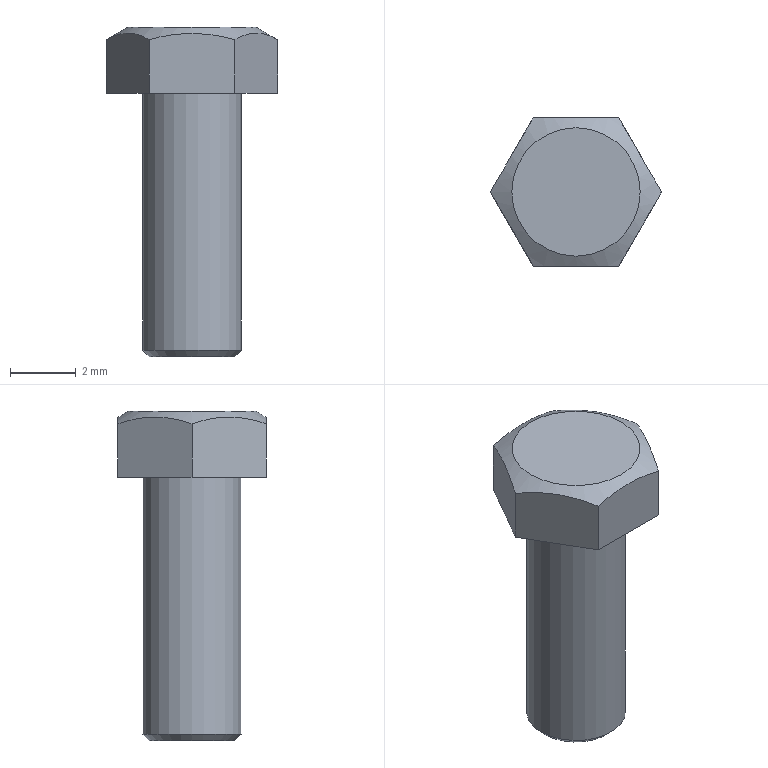Component | NX | SCREW_M3X8 | 1 solid | 12 faces | box 5.2 x 4.5 x 10 mm | volume 91 mm3 | plane 9 | cone 2 | cylinder 1 | commonest cylinder face diameters 3 x1
STEP:
#1=CARTESIAN_POINT('',(0.,0.,0.));
#2=DIRECTION('',(0.,0.,1.));
#3=DIRECTION('',(1.,0.,0.));
#4=AXIS2_PLACEMENT_3D('',#1,#2,#3);
#5=CARTESIAN_POINT('',(42.58,-10.,4.));
#6=VERTEX_POINT('',#5);
#7=CARTESIAN_POINT('',(43.88,-10.,4.));
#8=DIRECTION('',(0.,0.,-1.));
#9=DIRECTION('',(-1.,0.,0.));
#10=AXIS2_PLACEMENT_3D('',#7,#8,#9);
#11=CIRCLE('',#10,1.3);
#12=CARTESIAN_POINT('',(43.88,-10.,4.));
#13=DIRECTION('',(0.,0.,-1.));
#14=DIRECTION('',(-1.,0.,0.));
#15=AXIS2_PLACEMENT_3D('',#12,#13,#14);
#16=PLANE('',#15);
#17=CARTESIAN_POINT('',(0.,0.));
#18=DIRECTION('',(1.,0.));
#19=AXIS2_PLACEMENT_2D('',#17,#18);
#20=CIRCLE('',#19,1.3);
#21=(GEOMETRIC_REPRESENTATION_CONTEXT(2)PARAMETRIC_REPRESENTATION_CONTEXT()REPRESENTATION_CONTEXT('',''));
#22=DEFINITIONAL_REPRESENTATION('',(#20),#21);
#23=PCURVE('',#16,#22);
#24=CARTESIAN_POINT('',(43.88,-10.,4.2));
#25=DIRECTION('',(0.,0.,1.));
#26=DIRECTION('',(1.,0.,0.));
#27=AXIS2_PLACEMENT_3D('',#24,#25,#26);
#28=CONICAL_SURFACE('',#27,1.5,0.7854);
#29=CARTESIAN_POINT('',(9.425,-0.2));
#30=DIRECTION('',(-1.,0.));
#31=VECTOR('',#30,1.);
#32=LINE('',#29,#31);
#33=(GEOMETRIC_REPRESENTATION_CONTEXT(2)PARAMETRIC_REPRESENTATION_CONTEXT()REPRESENTATION_CONTEXT('',''));
#34=DEFINITIONAL_REPRESENTATION('',(#32),#33);
#35=PCURVE('',#28,#34);
#36=SURFACE_CURVE('',#11,(#23,#35),.PCURVE_S1.);
#37=EDGE_CURVE('',#6,#6,#36,.T.);
#38=ORIENTED_EDGE('',*,*,#37,.T.);
#39=EDGE_LOOP('',(#38));
#40=FACE_BOUND('',#39,.T.);
#41=ADVANCED_FACE('',(#40),#16,.T.);
#42=CARTESIAN_POINT('',(42.38,-10.,4.2));
#43=VERTEX_POINT('',#42);
#44=CARTESIAN_POINT('',(45.38,-10.,4.2));
#45=VERTEX_POINT('',#44);
#46=CARTESIAN_POINT('',(43.88,-10.,4.2));
#47=DIRECTION('',(0.,0.,1.));
#48=DIRECTION('',(-1.,0.,0.));
#49=AXIS2_PLACEMENT_3D('',#46,#47,#48);
#50=CIRCLE('',#49,1.5);
#51=CARTESIAN_POINT('',(43.88,-10.,4.));
#52=DIRECTION('',(0.,0.,1.));
#53=DIRECTION('',(1.,0.,0.));
#54=AXIS2_PLACEMENT_3D('',#51,#52,#53);
#55=CYLINDRICAL_SURFACE('',#54,1.5);
#56=CARTESIAN_POINT('',(3.142,0.2));
#57=DIRECTION('',(1.,0.));
#58=VECTOR('',#57,1.);
#59=LINE('',#56,#58);
#60=(GEOMETRIC_REPRESENTATION_CONTEXT(2)PARAMETRIC_REPRESENTATION_CONTEXT()REPRESENTATION_CONTEXT('',''));
#61=DEFINITIONAL_REPRESENTATION('',(#59),#60);
#62=PCURVE('',#55,#61);
#63=CARTESIAN_POINT('',(3.142,0.));
#64=DIRECTION('',(1.,0.));
#65=VECTOR('',#64,1.);
#66=LINE('',#63,#65);
#67=(GEOMETRIC_REPRESENTATION_CONTEXT(2)PARAMETRIC_REPRESENTATION_CONTEXT()REPRESENTATION_CONTEXT('',''));
#68=DEFINITIONAL_REPRESENTATION('',(#66),#67);
#69=PCURVE('',#28,#68);
#70=SURFACE_CURVE('',#50,(#62,#69),.PCURVE_S1.);
#71=EDGE_CURVE('',#43,#45,#70,.T.);
#72=ORIENTED_EDGE('',*,*,#71,.T.);
#73=CARTESIAN_POINT('',(45.38,-10.,12.));
#74=VERTEX_POINT('',#73);
#75=CARTESIAN_POINT('',(45.38,-10.,4.2));
#76=CARTESIAN_POINT('',(45.38,-10.,12.));
#77=B_SPLINE_CURVE_WITH_KNOTS('',1,(#75,#76),.UNSPECIFIED.,.F.,.F.,(2,2),(0.2,8.),.PIECEWISE_BEZIER_KNOTS.);
#78=CARTESIAN_POINT('',(6.283,0.));
#79=DIRECTION('',(0.,1.));
#80=VECTOR('',#79,1.);
#81=LINE('',#78,#80);
#82=(GEOMETRIC_REPRESENTATION_CONTEXT(2)PARAMETRIC_REPRESENTATION_CONTEXT()REPRESENTATION_CONTEXT('',''));
#83=DEFINITIONAL_REPRESENTATION('',(#81),#82);
#84=PCURVE('',#55,#83);
#85=CARTESIAN_POINT('',(0.,0.));
#86=DIRECTION('',(0.,1.));
#87=VECTOR('',#86,1.);
#88=LINE('',#85,#87);
#89=(GEOMETRIC_REPRESENTATION_CONTEXT(2)PARAMETRIC_REPRESENTATION_CONTEXT()REPRESENTATION_CONTEXT('',''));
#90=DEFINITIONAL_REPRESENTATION('',(#88),#89);
#91=PCURVE('',#55,#90);
#92=SEAM_CURVE('',#77,(#84,#91),.PCURVE_S1.);
#93=EDGE_CURVE('',#45,#74,#92,.T.);
#94=ORIENTED_EDGE('',*,*,#93,.T.);
#95=CARTESIAN_POINT('',(43.88,-10.,12.));
#96=DIRECTION('',(0.,0.,-1.));
#97=DIRECTION('',(1.,0.,0.));
#98=AXIS2_PLACEMENT_3D('',#95,#96,#97);
#99=CIRCLE('',#98,1.5);
#100=CARTESIAN_POINT('',(6.283,8.));
#101=DIRECTION('',(-1.,0.));
#102=VECTOR('',#101,1.);
#103=LINE('',#100,#102);
#104=(GEOMETRIC_REPRESENTATION_CONTEXT(2)PARAMETRIC_REPRESENTATION_CONTEXT()REPRESENTATION_CONTEXT('',''));
#105=DEFINITIONAL_REPRESENTATION('',(#103),#104);
#106=PCURVE('',#55,#105);
#107=CARTESIAN_POINT('',(43.88,-10.,12.));
#108=DIRECTION('',(0.,0.,-1.));
#109=DIRECTION('',(-1.,0.,0.));
#110=AXIS2_PLACEMENT_3D('',#107,#108,#109);
#111=PLANE('',#110);
#112=CARTESIAN_POINT('',(0.,0.));
#113=DIRECTION('',(-1.,0.));
#114=AXIS2_PLACEMENT_2D('',#112,#113);
#115=CIRCLE('',#114,1.5);
#116=(GEOMETRIC_REPRESENTATION_CONTEXT(2)PARAMETRIC_REPRESENTATION_CONTEXT()REPRESENTATION_CONTEXT('',''));
#117=DEFINITIONAL_REPRESENTATION('',(#115),#116);
#118=PCURVE('',#111,#117);
#119=SURFACE_CURVE('',#99,(#106,#118),.PCURVE_S1.);
#120=EDGE_CURVE('',#74,#74,#119,.T.);
#121=ORIENTED_EDGE('',*,*,#120,.T.);
#122=ORIENTED_EDGE('',*,*,#93,.F.);
#123=CARTESIAN_POINT('',(43.88,-10.,4.2));
#124=DIRECTION('',(0.,0.,1.));
#125=DIRECTION('',(-1.,0.,0.));
#126=AXIS2_PLACEMENT_3D('',#123,#124,#125);
#127=CIRCLE('',#126,1.5);
#128=CARTESIAN_POINT('',(-3.142,0.2));
#129=DIRECTION('',(1.,0.));
#130=VECTOR('',#129,1.);
#131=LINE('',#128,#130);
#132=(GEOMETRIC_REPRESENTATION_CONTEXT(2)PARAMETRIC_REPRESENTATION_CONTEXT()REPRESENTATION_CONTEXT('',''));
#133=DEFINITIONAL_REPRESENTATION('',(#131),#132);
#134=PCURVE('',#55,#133);
#135=CARTESIAN_POINT('',(3.142,0.));
#136=DIRECTION('',(1.,0.));
#137=VECTOR('',#136,1.);
#138=LINE('',#135,#137);
#139=(GEOMETRIC_REPRESENTATION_CONTEXT(2)PARAMETRIC_REPRESENTATION_CONTEXT()REPRESENTATION_CONTEXT('',''));
#140=DEFINITIONAL_REPRESENTATION('',(#138),#139);
#141=PCURVE('',#28,#140);
#142=SURFACE_CURVE('',#127,(#134,#141),.PCURVE_S1.);
#143=EDGE_CURVE('',#45,#43,#142,.T.);
#144=ORIENTED_EDGE('',*,*,#143,.T.);
#145=EDGE_LOOP('',(#72,#94,#121,#122,#144));
#146=FACE_BOUND('',#145,.T.);
#147=ADVANCED_FACE('',(#146),#55,.T.);
#148=CARTESIAN_POINT('',(46.478,-10.,13.625));
#149=VERTEX_POINT('',#148);
#150=CARTESIAN_POINT('',(45.179,-7.75,13.625));
#151=VERTEX_POINT('',#150);
#152=CARTESIAN_POINT('',(46.478,-10.,13.625));
#153=CARTESIAN_POINT('',(46.253,-9.61,13.755));
#154=CARTESIAN_POINT('',(46.017,-9.201,13.836));
#155=CARTESIAN_POINT('',(45.782,-8.795,13.825));
#156=CARTESIAN_POINT('',(45.579,-8.442,13.815));
#157=CARTESIAN_POINT('',(45.375,-8.089,13.738));
#158=CARTESIAN_POINT('',(45.179,-7.75,13.625));
#159=B_SPLINE_CURVE_WITH_KNOTS('',3,(#152,#153,#154,#155,#156,#157,#158),.UNSPECIFIED.,.F.,.F.,(4,3,4),(0.,0.5357,1.),.UNSPECIFIED.);
#160=CARTESIAN_POINT('',(45.179,-7.75,14.));
#161=DIRECTION('',(0.866,0.5,0.));
#162=DIRECTION('',(-0.5,0.866,0.));
#163=AXIS2_PLACEMENT_3D('',#160,#161,#162);
#164=PLANE('',#163);
#165=CARTESIAN_POINT('',(-2.598,-0.375));
#166=CARTESIAN_POINT('',(-2.148,-0.2451));
#167=CARTESIAN_POINT('',(-1.675,-0.1641));
#168=CARTESIAN_POINT('',(-1.207,-0.1751));
#169=CARTESIAN_POINT('',(-0.7992,-0.1848));
#170=CARTESIAN_POINT('',(-0.3917,-0.2619));
#171=CARTESIAN_POINT('',(0.,-0.375));
#172=B_SPLINE_CURVE_WITH_KNOTS('',3,(#165,#166,#167,#168,#169,#170,#171),.UNSPECIFIED.,.F.,.F.,(4,3,4),(0.,0.5357,1.),.UNSPECIFIED.);
#173=(GEOMETRIC_REPRESENTATION_CONTEXT(2)PARAMETRIC_REPRESENTATION_CONTEXT()REPRESENTATION_CONTEXT('',''));
#174=DEFINITIONAL_REPRESENTATION('',(#172),#173);
#175=PCURVE('',#164,#174);
#176=CARTESIAN_POINT('',(43.88,-10.,14.));
#177=DIRECTION('',(0.,0.,-1.));
#178=DIRECTION('',(-1.,0.,0.));
#179=AXIS2_PLACEMENT_3D('',#176,#177,#178);
#180=CONICAL_SURFACE('',#179,1.949,1.047);
#181=CARTESIAN_POINT('',(3.142,0.375));
#182=CARTESIAN_POINT('',(3.129,0.364));
#183=CARTESIAN_POINT('',(3.103,0.3426));
#184=CARTESIAN_POINT('',(3.062,0.3126));
#185=CARTESIAN_POINT('',(3.018,0.2851));
#186=CARTESIAN_POINT('',(2.973,0.2601));
#187=CARTESIAN_POINT('',(2.926,0.238));
#188=CARTESIAN_POINT('',(2.878,0.2188));
#189=CARTESIAN_POINT('',(2.828,0.2028));
#190=CARTESIAN_POINT('',(2.777,0.1902));
#191=CARTESIAN_POINT('',(2.724,0.181));
#192=CARTESIAN_POINT('',(2.672,0.1754));
#193=CARTESIAN_POINT('',(2.619,0.1734));
#194=CARTESIAN_POINT('',(2.566,0.1752));
#195=CARTESIAN_POINT('',(2.513,0.1807));
#196=CARTESIAN_POINT('',(2.46,0.1898));
#197=CARTESIAN_POINT('',(2.409,0.2024));
#198=CARTESIAN_POINT('',(2.359,0.2184));
#199=CARTESIAN_POINT('',(2.31,0.2376));
#200=CARTESIAN_POINT('',(2.263,0.2598));
#201=CARTESIAN_POINT('',(2.218,0.2848));
#202=CARTESIAN_POINT('',(2.175,0.3124));
#203=CARTESIAN_POINT('',(2.133,0.3424));
#204=CARTESIAN_POINT('',(2.107,0.3639));
#205=CARTESIAN_POINT('',(2.094,0.375));
#206=B_SPLINE_CURVE_WITH_KNOTS('',3,(#181,#182,#183,#184,#185,#186,#187,#188,#189,#190,#191,#192,#193,#194,#195,#196,#197,#198,#199,#200,#201,#202,#203,#204,#205),.UNSPECIFIED.,.F.,.F.,(4,1,1,1,1,1,1,1,1,1,1,1,1,1,1,1,1,1,1,1,1,1,4),(0.,0.04545,0.09091,0.1364,0.1818,0.2273,0.2727,0.3182,0.3636,0.4091,0.4545,0.5,0.5455,0.5909,0.6364,0.6818,0.7273,0.7727,0.8182,0.8636,0.9091,0.9545,1.),.QUASI_UNIFORM_KNOTS.);
#207=(GEOMETRIC_REPRESENTATION_CONTEXT(2)PARAMETRIC_REPRESENTATION_CONTEXT()REPRESENTATION_CONTEXT('',''));
#208=DEFINITIONAL_REPRESENTATION('',(#206),#207);
#209=PCURVE('',#180,#208);
#210=SURFACE_CURVE('',#159,(#175,#209),.PCURVE_S1.);
#211=EDGE_CURVE('',#149,#151,#210,.T.);
#212=ORIENTED_EDGE('',*,*,#211,.F.);
#213=CARTESIAN_POINT('',(46.478,-10.,12.));
#214=VERTEX_POINT('',#213);
#215=CARTESIAN_POINT('',(46.478,-10.,14.));
#216=DIRECTION('',(0.,0.,-1.));
#217=VECTOR('',#216,1.);
#218=LINE('',#215,#217);
#219=CARTESIAN_POINT('',(-2.598,0.));
#220=DIRECTION('',(0.,-1.));
#221=VECTOR('',#220,1.);
#222=LINE('',#219,#221);
#223=(GEOMETRIC_REPRESENTATION_CONTEXT(2)PARAMETRIC_REPRESENTATION_CONTEXT()REPRESENTATION_CONTEXT('',''));
#224=DEFINITIONAL_REPRESENTATION('',(#222),#223);
#225=PCURVE('',#164,#224);
#226=CARTESIAN_POINT('',(46.478,-10.,14.));
#227=DIRECTION('',(0.866,-0.5,0.));
#228=DIRECTION('',(0.5,0.866,0.));
#229=AXIS2_PLACEMENT_3D('',#226,#227,#228);
#230=PLANE('',#229);
#231=CARTESIAN_POINT('',(0.,0.));
#232=DIRECTION('',(0.,-1.));
#233=VECTOR('',#232,1.);
#234=LINE('',#231,#233);
#235=(GEOMETRIC_REPRESENTATION_CONTEXT(2)PARAMETRIC_REPRESENTATION_CONTEXT()REPRESENTATION_CONTEXT('',''));
#236=DEFINITIONAL_REPRESENTATION('',(#234),#235);
#237=PCURVE('',#230,#236);
#238=SURFACE_CURVE('',#218,(#225,#237),.PCURVE_S1.);
#239=EDGE_CURVE('',#149,#214,#238,.T.);
#240=ORIENTED_EDGE('',*,*,#239,.T.);
#241=CARTESIAN_POINT('',(45.179,-7.75,12.));
#242=VERTEX_POINT('',#241);
#243=CARTESIAN_POINT('',(45.179,-7.75,12.));
#244=DIRECTION('',(0.5,-0.866,0.));
#245=VECTOR('',#244,1.);
#246=LINE('',#243,#245);
#247=CARTESIAN_POINT('',(0.,-2.));
#248=DIRECTION('',(-1.,0.));
#249=VECTOR('',#248,1.);
#250=LINE('',#247,#249);
#251=(GEOMETRIC_REPRESENTATION_CONTEXT(2)PARAMETRIC_REPRESENTATION_CONTEXT()REPRESENTATION_CONTEXT('',''));
#252=DEFINITIONAL_REPRESENTATION('',(#250),#251);
#253=PCURVE('',#164,#252);
#254=CARTESIAN_POINT('',(-1.299,2.25));
#255=DIRECTION('',(-0.5,-0.866));
#256=VECTOR('',#255,1.);
#257=LINE('',#254,#256);
#258=(GEOMETRIC_REPRESENTATION_CONTEXT(2)PARAMETRIC_REPRESENTATION_CONTEXT()REPRESENTATION_CONTEXT('',''));
#259=DEFINITIONAL_REPRESENTATION('',(#257),#258);
#260=PCURVE('',#111,#259);
#261=SURFACE_CURVE('',#246,(#253,#260),.PCURVE_S1.);
#262=EDGE_CURVE('',#242,#214,#261,.T.);
#263=ORIENTED_EDGE('',*,*,#262,.F.);
#264=CARTESIAN_POINT('',(45.179,-7.75,14.));
#265=DIRECTION('',(0.,0.,-1.));
#266=VECTOR('',#265,1.);
#267=LINE('',#264,#266);
#268=CARTESIAN_POINT('',(0.,0.));
#269=DIRECTION('',(0.,-1.));
#270=VECTOR('',#269,1.);
#271=LINE('',#268,#270);
#272=(GEOMETRIC_REPRESENTATION_CONTEXT(2)PARAMETRIC_REPRESENTATION_CONTEXT()REPRESENTATION_CONTEXT('',''));
#273=DEFINITIONAL_REPRESENTATION('',(#271),#272);
#274=PCURVE('',#164,#273);
#275=CARTESIAN_POINT('',(42.581,-7.75,14.));
#276=DIRECTION('',(0.,1.,0.));
#277=DIRECTION('',(-1.,0.,0.));
#278=AXIS2_PLACEMENT_3D('',#275,#276,#277);
#279=PLANE('',#278);
#280=CARTESIAN_POINT('',(-2.598,0.));
#281=DIRECTION('',(0.,-1.));
#282=VECTOR('',#281,1.);
#283=LINE('',#280,#282);
#284=(GEOMETRIC_REPRESENTATION_CONTEXT(2)PARAMETRIC_REPRESENTATION_CONTEXT()REPRESENTATION_CONTEXT('',''));
#285=DEFINITIONAL_REPRESENTATION('',(#283),#284);
#286=PCURVE('',#279,#285);
#287=SURFACE_CURVE('',#267,(#274,#286),.PCURVE_S1.);
#288=EDGE_CURVE('',#151,#242,#287,.T.);
#289=ORIENTED_EDGE('',*,*,#288,.F.);
#290=EDGE_LOOP('',(#212,#240,#263,#289));
#291=FACE_BOUND('',#290,.T.);
#292=ADVANCED_FACE('',(#291),#164,.T.);
#293=CARTESIAN_POINT('',(45.179,-12.25,13.625));
#294=VERTEX_POINT('',#293);
#295=CARTESIAN_POINT('',(45.179,-12.25,13.625));
#296=CARTESIAN_POINT('',(45.404,-11.86,13.755));
#297=CARTESIAN_POINT('',(45.64,-11.451,13.836));
#298=CARTESIAN_POINT('',(45.875,-11.045,13.825));
#299=CARTESIAN_POINT('',(46.078,-10.692,13.815));
#300=CARTESIAN_POINT('',(46.282,-10.339,13.738));
#301=CARTESIAN_POINT('',(46.478,-10.,13.625));
#302=B_SPLINE_CURVE_WITH_KNOTS('',3,(#295,#296,#297,#298,#299,#300,#301),.UNSPECIFIED.,.F.,.F.,(4,3,4),(0.,0.5357,1.),.UNSPECIFIED.);
#303=CARTESIAN_POINT('',(-2.598,-0.375));
#304=CARTESIAN_POINT('',(-2.148,-0.2451));
#305=CARTESIAN_POINT('',(-1.675,-0.1641));
#306=CARTESIAN_POINT('',(-1.207,-0.1751));
#307=CARTESIAN_POINT('',(-0.7992,-0.1848));
#308=CARTESIAN_POINT('',(-0.3917,-0.2619));
#309=CARTESIAN_POINT('',(0.,-0.375));
#310=B_SPLINE_CURVE_WITH_KNOTS('',3,(#303,#304,#305,#306,#307,#308,#309),.UNSPECIFIED.,.F.,.F.,(4,3,4),(0.,0.5357,1.),.UNSPECIFIED.);
#311=(GEOMETRIC_REPRESENTATION_CONTEXT(2)PARAMETRIC_REPRESENTATION_CONTEXT()REPRESENTATION_CONTEXT('',''));
#312=DEFINITIONAL_REPRESENTATION('',(#310),#311);
#313=PCURVE('',#230,#312);
#314=CARTESIAN_POINT('',(4.189,0.375));
#315=CARTESIAN_POINT('',(4.176,0.364));
#316=CARTESIAN_POINT('',(4.15,0.3426));
#317=CARTESIAN_POINT('',(4.109,0.3126));
#318=CARTESIAN_POINT('',(4.066,0.2851));
#319=CARTESIAN_POINT('',(4.02,0.2601));
#320=CARTESIAN_POINT('',(3.974,0.238));
#321=CARTESIAN_POINT('',(3.925,0.2188));
#322=CARTESIAN_POINT('',(3.875,0.2028));
#323=CARTESIAN_POINT('',(3.824,0.1902));
#324=CARTESIAN_POINT('',(3.772,0.181));
#325=CARTESIAN_POINT('',(3.719,0.1754));
#326=CARTESIAN_POINT('',(3.666,0.1734));
#327=CARTESIAN_POINT('',(3.613,0.1752));
#328=CARTESIAN_POINT('',(3.56,0.1807));
#329=CARTESIAN_POINT('',(3.508,0.1898));
#330=CARTESIAN_POINT('',(3.456,0.2024));
#331=CARTESIAN_POINT('',(3.406,0.2184));
#332=CARTESIAN_POINT('',(3.357,0.2376));
#333=CARTESIAN_POINT('',(3.31,0.2598));
#334=CARTESIAN_POINT('',(3.265,0.2848));
#335=CARTESIAN_POINT('',(3.222,0.3124));
#336=CARTESIAN_POINT('',(3.181,0.3424));
#337=CARTESIAN_POINT('',(3.154,0.3639));
#338=CARTESIAN_POINT('',(3.142,0.375));
#339=B_SPLINE_CURVE_WITH_KNOTS('',3,(#314,#315,#316,#317,#318,#319,#320,#321,#322,#323,#324,#325,#326,#327,#328,#329,#330,#331,#332,#333,#334,#335,#336,#337,#338),.UNSPECIFIED.,.F.,.F.,(4,1,1,1,1,1,1,1,1,1,1,1,1,1,1,1,1,1,1,1,1,1,4),(0.,0.04545,0.09091,0.1364,0.1818,0.2273,0.2727,0.3182,0.3636,0.4091,0.4545,0.5,0.5455,0.5909,0.6364,0.6818,0.7273,0.7727,0.8182,0.8636,0.9091,0.9545,1.),.QUASI_UNIFORM_KNOTS.);
#340=(GEOMETRIC_REPRESENTATION_CONTEXT(2)PARAMETRIC_REPRESENTATION_CONTEXT()REPRESENTATION_CONTEXT('',''));
#341=DEFINITIONAL_REPRESENTATION('',(#339),#340);
#342=PCURVE('',#180,#341);
#343=SURFACE_CURVE('',#302,(#313,#342),.PCURVE_S1.);
#344=EDGE_CURVE('',#294,#149,#343,.T.);
#345=ORIENTED_EDGE('',*,*,#344,.F.);
#346=CARTESIAN_POINT('',(45.179,-12.25,12.));
#347=VERTEX_POINT('',#346);
#348=CARTESIAN_POINT('',(45.179,-12.25,14.));
#349=DIRECTION('',(0.,0.,-1.));
#350=VECTOR('',#349,1.);
#351=LINE('',#348,#350);
#352=CARTESIAN_POINT('',(-2.598,0.));
#353=DIRECTION('',(0.,-1.));
#354=VECTOR('',#353,1.);
#355=LINE('',#352,#354);
#356=(GEOMETRIC_REPRESENTATION_CONTEXT(2)PARAMETRIC_REPRESENTATION_CONTEXT()REPRESENTATION_CONTEXT('',''));
#357=DEFINITIONAL_REPRESENTATION('',(#355),#356);
#358=PCURVE('',#230,#357);
#359=CARTESIAN_POINT('',(45.179,-12.25,14.));
#360=DIRECTION('',(0.,-1.,0.));
#361=DIRECTION('',(0.,0.,-1.));
#362=AXIS2_PLACEMENT_3D('',#359,#360,#361);
#363=PLANE('',#362);
#364=CARTESIAN_POINT('',(0.,0.));
#365=DIRECTION('',(1.,0.));
#366=VECTOR('',#365,1.);
#367=LINE('',#364,#366);
#368=(GEOMETRIC_REPRESENTATION_CONTEXT(2)PARAMETRIC_REPRESENTATION_CONTEXT()REPRESENTATION_CONTEXT('',''));
#369=DEFINITIONAL_REPRESENTATION('',(#367),#368);
#370=PCURVE('',#363,#369);
#371=SURFACE_CURVE('',#351,(#358,#370),.PCURVE_S1.);
#372=EDGE_CURVE('',#294,#347,#371,.T.);
#373=ORIENTED_EDGE('',*,*,#372,.T.);
#374=CARTESIAN_POINT('',(46.478,-10.,12.));
#375=DIRECTION('',(-0.5,-0.866,0.));
#376=VECTOR('',#375,1.);
#377=LINE('',#374,#376);
#378=CARTESIAN_POINT('',(0.,-2.));
#379=DIRECTION('',(-1.,0.));
#380=VECTOR('',#379,1.);
#381=LINE('',#378,#380);
#382=(GEOMETRIC_REPRESENTATION_CONTEXT(2)PARAMETRIC_REPRESENTATION_CONTEXT()REPRESENTATION_CONTEXT('',''));
#383=DEFINITIONAL_REPRESENTATION('',(#381),#382);
#384=PCURVE('',#230,#383);
#385=CARTESIAN_POINT('',(-2.598,0.));
#386=DIRECTION('',(0.5,-0.866));
#387=VECTOR('',#386,1.);
#388=LINE('',#385,#387);
#389=(GEOMETRIC_REPRESENTATION_CONTEXT(2)PARAMETRIC_REPRESENTATION_CONTEXT()REPRESENTATION_CONTEXT('',''));
#390=DEFINITIONAL_REPRESENTATION('',(#388),#389);
#391=PCURVE('',#111,#390);
#392=SURFACE_CURVE('',#377,(#384,#391),.PCURVE_S1.);
#393=EDGE_CURVE('',#214,#347,#392,.T.);
#394=ORIENTED_EDGE('',*,*,#393,.F.);
#395=ORIENTED_EDGE('',*,*,#239,.F.);
#396=EDGE_LOOP('',(#345,#373,#394,#395));
#397=FACE_BOUND('',#396,.T.);
#398=ADVANCED_FACE('',(#397),#230,.T.);
#399=CARTESIAN_POINT('',(42.581,-12.25,13.625));
#400=VERTEX_POINT('',#399);
#401=CARTESIAN_POINT('',(42.581,-12.25,13.625));
#402=CARTESIAN_POINT('',(43.426,-12.25,13.869));
#403=CARTESIAN_POINT('',(44.339,-12.25,13.867));
#404=CARTESIAN_POINT('',(45.179,-12.25,13.625));
#405=B_SPLINE_CURVE_WITH_KNOTS('',3,(#401,#402,#403,#404),.UNSPECIFIED.,.F.,.F.,(4,4),(0.,1.),.PIECEWISE_BEZIER_KNOTS.);
#406=CARTESIAN_POINT('',(0.375,-2.598));
#407=CARTESIAN_POINT('',(0.1311,-1.753));
#408=CARTESIAN_POINT('',(0.1325,-0.8399));
#409=CARTESIAN_POINT('',(0.375,0.));
#410=B_SPLINE_CURVE_WITH_KNOTS('',3,(#406,#407,#408,#409),.UNSPECIFIED.,.F.,.F.,(4,4),(0.,1.),.PIECEWISE_BEZIER_KNOTS.);
#411=(GEOMETRIC_REPRESENTATION_CONTEXT(2)PARAMETRIC_REPRESENTATION_CONTEXT()REPRESENTATION_CONTEXT('',''));
#412=DEFINITIONAL_REPRESENTATION('',(#410),#411);
#413=PCURVE('',#363,#412);
#414=CARTESIAN_POINT('',(5.236,0.375));
#415=CARTESIAN_POINT('',(5.223,0.3639));
#416=CARTESIAN_POINT('',(5.197,0.3425));
#417=CARTESIAN_POINT('',(5.156,0.3127));
#418=CARTESIAN_POINT('',(5.112,0.2856));
#419=CARTESIAN_POINT('',(5.067,0.2611));
#420=CARTESIAN_POINT('',(5.02,0.2396));
#421=CARTESIAN_POINT('',(4.971,0.221));
#422=CARTESIAN_POINT('',(4.921,0.2057));
#423=CARTESIAN_POINT('',(4.87,0.1937));
#424=CARTESIAN_POINT('',(4.818,0.185));
#425=CARTESIAN_POINT('',(4.765,0.1798));
#426=CARTESIAN_POINT('',(4.712,0.1781));
#427=CARTESIAN_POINT('',(4.658,0.1799));
#428=CARTESIAN_POINT('',(4.606,0.1852));
#429=CARTESIAN_POINT('',(4.553,0.194));
#430=CARTESIAN_POINT('',(4.502,0.2061));
#431=CARTESIAN_POINT('',(4.452,0.2215));
#432=CARTESIAN_POINT('',(4.404,0.24));
#433=CARTESIAN_POINT('',(4.357,0.2616));
#434=CARTESIAN_POINT('',(4.312,0.286));
#435=CARTESIAN_POINT('',(4.269,0.3131));
#436=CARTESIAN_POINT('',(4.228,0.3427));
#437=CARTESIAN_POINT('',(4.202,0.364));
#438=CARTESIAN_POINT('',(4.189,0.375));
#439=B_SPLINE_CURVE_WITH_KNOTS('',3,(#414,#415,#416,#417,#418,#419,#420,#421,#422,#423,#424,#425,#426,#427,#428,#429,#430,#431,#432,#433,#434,#435,#436,#437,#438),.UNSPECIFIED.,.F.,.F.,(4,1,1,1,1,1,1,1,1,1,1,1,1,1,1,1,1,1,1,1,1,1,4),(0.,0.04545,0.09091,0.1364,0.1818,0.2273,0.2727,0.3182,0.3636,0.4091,0.4545,0.5,0.5455,0.5909,0.6364,0.6818,0.7273,0.7727,0.8182,0.8636,0.9091,0.9545,1.),.QUASI_UNIFORM_KNOTS.);
#440=(GEOMETRIC_REPRESENTATION_CONTEXT(2)PARAMETRIC_REPRESENTATION_CONTEXT()REPRESENTATION_CONTEXT('',''));
#441=DEFINITIONAL_REPRESENTATION('',(#439),#440);
#442=PCURVE('',#180,#441);
#443=SURFACE_CURVE('',#405,(#413,#442),.PCURVE_S1.);
#444=EDGE_CURVE('',#400,#294,#443,.T.);
#445=ORIENTED_EDGE('',*,*,#444,.F.);
#446=CARTESIAN_POINT('',(42.581,-12.25,12.));
#447=VERTEX_POINT('',#446);
#448=CARTESIAN_POINT('',(42.581,-12.25,14.));
#449=DIRECTION('',(0.,0.,-1.));
#450=VECTOR('',#449,1.);
#451=LINE('',#448,#450);
#452=CARTESIAN_POINT('',(0.,-2.598));
#453=DIRECTION('',(1.,0.));
#454=VECTOR('',#453,1.);
#455=LINE('',#452,#454);
#456=(GEOMETRIC_REPRESENTATION_CONTEXT(2)PARAMETRIC_REPRESENTATION_CONTEXT()REPRESENTATION_CONTEXT('',''));
#457=DEFINITIONAL_REPRESENTATION('',(#455),#456);
#458=PCURVE('',#363,#457);
#459=CARTESIAN_POINT('',(42.581,-12.25,14.));
#460=DIRECTION('',(-0.866,-0.5,0.));
#461=DIRECTION('',(0.5,-0.866,0.));
#462=AXIS2_PLACEMENT_3D('',#459,#460,#461);
#463=PLANE('',#462);
#464=CARTESIAN_POINT('',(0.,0.));
#465=DIRECTION('',(0.,-1.));
#466=VECTOR('',#465,1.);
#467=LINE('',#464,#466);
#468=(GEOMETRIC_REPRESENTATION_CONTEXT(2)PARAMETRIC_REPRESENTATION_CONTEXT()REPRESENTATION_CONTEXT('',''));
#469=DEFINITIONAL_REPRESENTATION('',(#467),#468);
#470=PCURVE('',#463,#469);
#471=SURFACE_CURVE('',#451,(#458,#470),.PCURVE_S1.);
#472=EDGE_CURVE('',#400,#447,#471,.T.);
#473=ORIENTED_EDGE('',*,*,#472,.T.);
#474=CARTESIAN_POINT('',(45.179,-12.25,12.));
#475=DIRECTION('',(-1.,0.,0.));
#476=VECTOR('',#475,1.);
#477=LINE('',#474,#476);
#478=CARTESIAN_POINT('',(2.,0.));
#479=DIRECTION('',(0.,-1.));
#480=VECTOR('',#479,1.);
#481=LINE('',#478,#480);
#482=(GEOMETRIC_REPRESENTATION_CONTEXT(2)PARAMETRIC_REPRESENTATION_CONTEXT()REPRESENTATION_CONTEXT('',''));
#483=DEFINITIONAL_REPRESENTATION('',(#481),#482);
#484=PCURVE('',#363,#483);
#485=CARTESIAN_POINT('',(-1.299,-2.25));
#486=DIRECTION('',(1.,0.));
#487=VECTOR('',#486,1.);
#488=LINE('',#485,#487);
#489=(GEOMETRIC_REPRESENTATION_CONTEXT(2)PARAMETRIC_REPRESENTATION_CONTEXT()REPRESENTATION_CONTEXT('',''));
#490=DEFINITIONAL_REPRESENTATION('',(#488),#489);
#491=PCURVE('',#111,#490);
#492=SURFACE_CURVE('',#477,(#484,#491),.PCURVE_S1.);
#493=EDGE_CURVE('',#347,#447,#492,.T.);
#494=ORIENTED_EDGE('',*,*,#493,.F.);
#495=ORIENTED_EDGE('',*,*,#372,.F.);
#496=EDGE_LOOP('',(#445,#473,#494,#495));
#497=FACE_BOUND('',#496,.T.);
#498=ADVANCED_FACE('',(#497),#363,.T.);
#499=CARTESIAN_POINT('',(41.282,-10.,13.625));
#500=VERTEX_POINT('',#499);
#501=CARTESIAN_POINT('',(41.282,-10.,13.625));
#502=CARTESIAN_POINT('',(41.507,-10.39,13.755));
#503=CARTESIAN_POINT('',(41.743,-10.799,13.836));
#504=CARTESIAN_POINT('',(41.978,-11.205,13.825));
#505=CARTESIAN_POINT('',(42.181,-11.558,13.815));
#506=CARTESIAN_POINT('',(42.385,-11.911,13.738));
#507=CARTESIAN_POINT('',(42.581,-12.25,13.625));
#508=B_SPLINE_CURVE_WITH_KNOTS('',3,(#501,#502,#503,#504,#505,#506,#507),.UNSPECIFIED.,.F.,.F.,(4,3,4),(0.,0.5357,1.),.UNSPECIFIED.);
#509=CARTESIAN_POINT('',(-2.598,-0.375));
#510=CARTESIAN_POINT('',(-2.148,-0.2451));
#511=CARTESIAN_POINT('',(-1.675,-0.1641));
#512=CARTESIAN_POINT('',(-1.207,-0.1751));
#513=CARTESIAN_POINT('',(-0.7992,-0.1848));
#514=CARTESIAN_POINT('',(-0.3917,-0.2619));
#515=CARTESIAN_POINT('',(0.,-0.375));
#516=B_SPLINE_CURVE_WITH_KNOTS('',3,(#509,#510,#511,#512,#513,#514,#515),.UNSPECIFIED.,.F.,.F.,(4,3,4),(0.,0.5357,1.),.UNSPECIFIED.);
#517=(GEOMETRIC_REPRESENTATION_CONTEXT(2)PARAMETRIC_REPRESENTATION_CONTEXT()REPRESENTATION_CONTEXT('',''));
#518=DEFINITIONAL_REPRESENTATION('',(#516),#517);
#519=PCURVE('',#463,#518);
#520=CARTESIAN_POINT('',(6.283,0.375));
#521=CARTESIAN_POINT('',(6.27,0.364));
#522=CARTESIAN_POINT('',(6.244,0.3426));
#523=CARTESIAN_POINT('',(6.203,0.3126));
#524=CARTESIAN_POINT('',(6.16,0.2851));
#525=CARTESIAN_POINT('',(6.115,0.2601));
#526=CARTESIAN_POINT('',(6.068,0.238));
#527=CARTESIAN_POINT('',(6.019,0.2188));
#528=CARTESIAN_POINT('',(5.969,0.2028));
#529=CARTESIAN_POINT('',(5.918,0.1902));
#530=CARTESIAN_POINT('',(5.866,0.181));
#531=CARTESIAN_POINT('',(5.813,0.1754));
#532=CARTESIAN_POINT('',(5.76,0.1734));
#533=CARTESIAN_POINT('',(5.707,0.1752));
#534=CARTESIAN_POINT('',(5.654,0.1807));
#535=CARTESIAN_POINT('',(5.602,0.1898));
#536=CARTESIAN_POINT('',(5.551,0.2024));
#537=CARTESIAN_POINT('',(5.501,0.2184));
#538=CARTESIAN_POINT('',(5.452,0.2376));
#539=CARTESIAN_POINT('',(5.405,0.2598));
#540=CARTESIAN_POINT('',(5.36,0.2848));
#541=CARTESIAN_POINT('',(5.316,0.3124));
#542=CARTESIAN_POINT('',(5.275,0.3424));
#543=CARTESIAN_POINT('',(5.249,0.3639));
#544=CARTESIAN_POINT('',(5.236,0.375));
#545=B_SPLINE_CURVE_WITH_KNOTS('',3,(#520,#521,#522,#523,#524,#525,#526,#527,#528,#529,#530,#531,#532,#533,#534,#535,#536,#537,#538,#539,#540,#541,#542,#543,#544),.UNSPECIFIED.,.F.,.F.,(4,1,1,1,1,1,1,1,1,1,1,1,1,1,1,1,1,1,1,1,1,1,4),(0.,0.04545,0.09091,0.1364,0.1818,0.2273,0.2727,0.3182,0.3636,0.4091,0.4545,0.5,0.5455,0.5909,0.6364,0.6818,0.7273,0.7727,0.8182,0.8636,0.9091,0.9545,1.),.QUASI_UNIFORM_KNOTS.);
#546=(GEOMETRIC_REPRESENTATION_CONTEXT(2)PARAMETRIC_REPRESENTATION_CONTEXT()REPRESENTATION_CONTEXT('',''));
#547=DEFINITIONAL_REPRESENTATION('',(#545),#546);
#548=PCURVE('',#180,#547);
#549=SURFACE_CURVE('',#508,(#519,#548),.PCURVE_S1.);
#550=EDGE_CURVE('',#500,#400,#549,.T.);
#551=ORIENTED_EDGE('',*,*,#550,.F.);
#552=CARTESIAN_POINT('',(41.282,-10.,12.));
#553=VERTEX_POINT('',#552);
#554=CARTESIAN_POINT('',(41.282,-10.,14.));
#555=DIRECTION('',(0.,0.,-1.));
#556=VECTOR('',#555,1.);
#557=LINE('',#554,#556);
#558=CARTESIAN_POINT('',(-2.598,0.));
#559=DIRECTION('',(0.,-1.));
#560=VECTOR('',#559,1.);
#561=LINE('',#558,#560);
#562=(GEOMETRIC_REPRESENTATION_CONTEXT(2)PARAMETRIC_REPRESENTATION_CONTEXT()REPRESENTATION_CONTEXT('',''));
#563=DEFINITIONAL_REPRESENTATION('',(#561),#562);
#564=PCURVE('',#463,#563);
#565=CARTESIAN_POINT('',(41.282,-10.,14.));
#566=DIRECTION('',(-0.866,0.5,0.));
#567=DIRECTION('',(-0.5,-0.866,0.));
#568=AXIS2_PLACEMENT_3D('',#565,#566,#567);
#569=PLANE('',#568);
#570=CARTESIAN_POINT('',(0.,0.));
#571=DIRECTION('',(0.,-1.));
#572=VECTOR('',#571,1.);
#573=LINE('',#570,#572);
#574=(GEOMETRIC_REPRESENTATION_CONTEXT(2)PARAMETRIC_REPRESENTATION_CONTEXT()REPRESENTATION_CONTEXT('',''));
#575=DEFINITIONAL_REPRESENTATION('',(#573),#574);
#576=PCURVE('',#569,#575);
#577=SURFACE_CURVE('',#557,(#564,#576),.PCURVE_S1.);
#578=EDGE_CURVE('',#500,#553,#577,.T.);
#579=ORIENTED_EDGE('',*,*,#578,.T.);
#580=CARTESIAN_POINT('',(42.581,-12.25,12.));
#581=DIRECTION('',(-0.5,0.866,0.));
#582=VECTOR('',#581,1.);
#583=LINE('',#580,#582);
#584=CARTESIAN_POINT('',(0.,-2.));
#585=DIRECTION('',(-1.,0.));
#586=VECTOR('',#585,1.);
#587=LINE('',#584,#586);
#588=(GEOMETRIC_REPRESENTATION_CONTEXT(2)PARAMETRIC_REPRESENTATION_CONTEXT()REPRESENTATION_CONTEXT('',''));
#589=DEFINITIONAL_REPRESENTATION('',(#587),#588);
#590=PCURVE('',#463,#589);
#591=CARTESIAN_POINT('',(1.299,-2.25));
#592=DIRECTION('',(0.5,0.866));
#593=VECTOR('',#592,1.);
#594=LINE('',#591,#593);
#595=(GEOMETRIC_REPRESENTATION_CONTEXT(2)PARAMETRIC_REPRESENTATION_CONTEXT()REPRESENTATION_CONTEXT('',''));
#596=DEFINITIONAL_REPRESENTATION('',(#594),#595);
#597=PCURVE('',#111,#596);
#598=SURFACE_CURVE('',#583,(#590,#597),.PCURVE_S1.);
#599=EDGE_CURVE('',#447,#553,#598,.T.);
#600=ORIENTED_EDGE('',*,*,#599,.F.);
#601=ORIENTED_EDGE('',*,*,#472,.F.);
#602=EDGE_LOOP('',(#551,#579,#600,#601));
#603=FACE_BOUND('',#602,.T.);
#604=ADVANCED_FACE('',(#603),#463,.T.);
#605=CARTESIAN_POINT('',(42.581,-7.75,13.625));
#606=VERTEX_POINT('',#605);
#607=CARTESIAN_POINT('',(42.581,-7.75,13.625));
#608=CARTESIAN_POINT('',(42.356,-8.14,13.755));
#609=CARTESIAN_POINT('',(42.12,-8.549,13.836));
#610=CARTESIAN_POINT('',(41.885,-8.955,13.825));
#611=CARTESIAN_POINT('',(41.682,-9.308,13.815));
#612=CARTESIAN_POINT('',(41.478,-9.661,13.738));
#613=CARTESIAN_POINT('',(41.282,-10.,13.625));
#614=B_SPLINE_CURVE_WITH_KNOTS('',3,(#607,#608,#609,#610,#611,#612,#613),.UNSPECIFIED.,.F.,.F.,(4,3,4),(0.,0.5357,1.),.UNSPECIFIED.);
#615=CARTESIAN_POINT('',(-2.598,-0.375));
#616=CARTESIAN_POINT('',(-2.148,-0.2451));
#617=CARTESIAN_POINT('',(-1.675,-0.1641));
#618=CARTESIAN_POINT('',(-1.207,-0.1751));
#619=CARTESIAN_POINT('',(-0.7992,-0.1848));
#620=CARTESIAN_POINT('',(-0.3917,-0.2619));
#621=CARTESIAN_POINT('',(0.,-0.375));
#622=B_SPLINE_CURVE_WITH_KNOTS('',3,(#615,#616,#617,#618,#619,#620,#621),.UNSPECIFIED.,.F.,.F.,(4,3,4),(0.,0.5357,1.),.UNSPECIFIED.);
#623=(GEOMETRIC_REPRESENTATION_CONTEXT(2)PARAMETRIC_REPRESENTATION_CONTEXT()REPRESENTATION_CONTEXT('',''));
#624=DEFINITIONAL_REPRESENTATION('',(#622),#623);
#625=PCURVE('',#569,#624);
#626=CARTESIAN_POINT('',(1.047,0.375));
#627=CARTESIAN_POINT('',(1.034,0.364));
#628=CARTESIAN_POINT('',(1.008,0.3426));
#629=CARTESIAN_POINT('',(0.9671,0.3126));
#630=CARTESIAN_POINT('',(0.9239,0.2851));
#631=CARTESIAN_POINT('',(0.8788,0.2601));
#632=CARTESIAN_POINT('',(0.8319,0.238));
#633=CARTESIAN_POINT('',(0.7834,0.2188));
#634=CARTESIAN_POINT('',(0.7334,0.2028));
#635=CARTESIAN_POINT('',(0.6822,0.1902));
#636=CARTESIAN_POINT('',(0.63,0.181));
#637=CARTESIAN_POINT('',(0.5773,0.1754));
#638=CARTESIAN_POINT('',(0.5242,0.1734));
#639=CARTESIAN_POINT('',(0.4712,0.1752));
#640=CARTESIAN_POINT('',(0.4182,0.1807));
#641=CARTESIAN_POINT('',(0.366,0.1898));
#642=CARTESIAN_POINT('',(0.3147,0.2024));
#643=CARTESIAN_POINT('',(0.2646,0.2184));
#644=CARTESIAN_POINT('',(0.2159,0.2376));
#645=CARTESIAN_POINT('',(0.1689,0.2598));
#646=CARTESIAN_POINT('',(0.1237,0.2848));
#647=CARTESIAN_POINT('',(0.08036,0.3124));
#648=CARTESIAN_POINT('',(0.03902,0.3424));
#649=CARTESIAN_POINT('',(0.01278,0.3639));
#650=CARTESIAN_POINT('',(0.,0.375));
#651=B_SPLINE_CURVE_WITH_KNOTS('',3,(#626,#627,#628,#629,#630,#631,#632,#633,#634,#635,#636,#637,#638,#639,#640,#641,#642,#643,#644,#645,#646,#647,#648,#649,#650),.UNSPECIFIED.,.F.,.F.,(4,1,1,1,1,1,1,1,1,1,1,1,1,1,1,1,1,1,1,1,1,1,4),(0.,0.04545,0.09091,0.1364,0.1818,0.2273,0.2727,0.3182,0.3636,0.4091,0.4545,0.5,0.5455,0.5909,0.6364,0.6818,0.7273,0.7727,0.8182,0.8636,0.9091,0.9545,1.),.QUASI_UNIFORM_KNOTS.);
#652=(GEOMETRIC_REPRESENTATION_CONTEXT(2)PARAMETRIC_REPRESENTATION_CONTEXT()REPRESENTATION_CONTEXT('',''));
#653=DEFINITIONAL_REPRESENTATION('',(#651),#652);
#654=PCURVE('',#180,#653);
#655=SURFACE_CURVE('',#614,(#625,#654),.PCURVE_S1.);
#656=EDGE_CURVE('',#606,#500,#655,.T.);
#657=ORIENTED_EDGE('',*,*,#656,.F.);
#658=CARTESIAN_POINT('',(42.581,-7.75,12.));
#659=VERTEX_POINT('',#658);
#660=CARTESIAN_POINT('',(42.581,-7.75,14.));
#661=DIRECTION('',(0.,0.,-1.));
#662=VECTOR('',#661,1.);
#663=LINE('',#660,#662);
#664=CARTESIAN_POINT('',(-2.598,0.));
#665=DIRECTION('',(0.,-1.));
#666=VECTOR('',#665,1.);
#667=LINE('',#664,#666);
#668=(GEOMETRIC_REPRESENTATION_CONTEXT(2)PARAMETRIC_REPRESENTATION_CONTEXT()REPRESENTATION_CONTEXT('',''));
#669=DEFINITIONAL_REPRESENTATION('',(#667),#668);
#670=PCURVE('',#569,#669);
#671=CARTESIAN_POINT('',(0.,0.));
#672=DIRECTION('',(0.,-1.));
#673=VECTOR('',#672,1.);
#674=LINE('',#671,#673);
#675=(GEOMETRIC_REPRESENTATION_CONTEXT(2)PARAMETRIC_REPRESENTATION_CONTEXT()REPRESENTATION_CONTEXT('',''));
#676=DEFINITIONAL_REPRESENTATION('',(#674),#675);
#677=PCURVE('',#279,#676);
#678=SURFACE_CURVE('',#663,(#670,#677),.PCURVE_S1.);
#679=EDGE_CURVE('',#606,#659,#678,.T.);
#680=ORIENTED_EDGE('',*,*,#679,.T.);
#681=CARTESIAN_POINT('',(41.282,-10.,12.));
#682=DIRECTION('',(0.5,0.866,0.));
#683=VECTOR('',#682,1.);
#684=LINE('',#681,#683);
#685=CARTESIAN_POINT('',(0.,-2.));
#686=DIRECTION('',(-1.,0.));
#687=VECTOR('',#686,1.);
#688=LINE('',#685,#687);
#689=(GEOMETRIC_REPRESENTATION_CONTEXT(2)PARAMETRIC_REPRESENTATION_CONTEXT()REPRESENTATION_CONTEXT('',''));
#690=DEFINITIONAL_REPRESENTATION('',(#688),#689);
#691=PCURVE('',#569,#690);
#692=CARTESIAN_POINT('',(2.598,0.));
#693=DIRECTION('',(-0.5,0.866));
#694=VECTOR('',#693,1.);
#695=LINE('',#692,#694);
#696=(GEOMETRIC_REPRESENTATION_CONTEXT(2)PARAMETRIC_REPRESENTATION_CONTEXT()REPRESENTATION_CONTEXT('',''));
#697=DEFINITIONAL_REPRESENTATION('',(#695),#696);
#698=PCURVE('',#111,#697);
#699=SURFACE_CURVE('',#684,(#691,#698),.PCURVE_S1.);
#700=EDGE_CURVE('',#553,#659,#699,.T.);
#701=ORIENTED_EDGE('',*,*,#700,.F.);
#702=ORIENTED_EDGE('',*,*,#578,.F.);
#703=EDGE_LOOP('',(#657,#680,#701,#702));
#704=FACE_BOUND('',#703,.T.);
#705=ADVANCED_FACE('',(#704),#569,.T.);
#706=CARTESIAN_POINT('',(45.179,-7.75,13.625));
#707=CARTESIAN_POINT('',(44.339,-7.75,13.867));
#708=CARTESIAN_POINT('',(43.426,-7.75,13.869));
#709=CARTESIAN_POINT('',(42.581,-7.75,13.625));
#710=B_SPLINE_CURVE_WITH_KNOTS('',3,(#706,#707,#708,#709),.UNSPECIFIED.,.F.,.F.,(4,4),(0.,1.),.PIECEWISE_BEZIER_KNOTS.);
#711=CARTESIAN_POINT('',(-2.598,-0.375));
#712=CARTESIAN_POINT('',(-1.758,-0.1325));
#713=CARTESIAN_POINT('',(-0.845,-0.1311));
#714=CARTESIAN_POINT('',(0.,-0.375));
#715=B_SPLINE_CURVE_WITH_KNOTS('',3,(#711,#712,#713,#714),.UNSPECIFIED.,.F.,.F.,(4,4),(0.,1.),.PIECEWISE_BEZIER_KNOTS.);
#716=(GEOMETRIC_REPRESENTATION_CONTEXT(2)PARAMETRIC_REPRESENTATION_CONTEXT()REPRESENTATION_CONTEXT('',''));
#717=DEFINITIONAL_REPRESENTATION('',(#715),#716);
#718=PCURVE('',#279,#717);
#719=CARTESIAN_POINT('',(2.094,0.375));
#720=CARTESIAN_POINT('',(2.082,0.364));
#721=CARTESIAN_POINT('',(2.056,0.3427));
#722=CARTESIAN_POINT('',(2.014,0.3131));
#723=CARTESIAN_POINT('',(1.971,0.286));
#724=CARTESIAN_POINT('',(1.926,0.2616));
#725=CARTESIAN_POINT('',(1.879,0.24));
#726=CARTESIAN_POINT('',(1.831,0.2215));
#727=CARTESIAN_POINT('',(1.781,0.2061));
#728=CARTESIAN_POINT('',(1.73,0.194));
#729=CARTESIAN_POINT('',(1.678,0.1852));
#730=CARTESIAN_POINT('',(1.625,0.1799));
#731=CARTESIAN_POINT('',(1.572,0.1781));
#732=CARTESIAN_POINT('',(1.518,0.1798));
#733=CARTESIAN_POINT('',(1.466,0.185));
#734=CARTESIAN_POINT('',(1.413,0.1937));
#735=CARTESIAN_POINT('',(1.362,0.2057));
#736=CARTESIAN_POINT('',(1.312,0.221));
#737=CARTESIAN_POINT('',(1.263,0.2396));
#738=CARTESIAN_POINT('',(1.216,0.2611));
#739=CARTESIAN_POINT('',(1.171,0.2856));
#740=CARTESIAN_POINT('',(1.128,0.3127));
#741=CARTESIAN_POINT('',(1.086,0.3425));
#742=CARTESIAN_POINT('',(1.06,0.3639));
#743=CARTESIAN_POINT('',(1.047,0.375));
#744=B_SPLINE_CURVE_WITH_KNOTS('',3,(#719,#720,#721,#722,#723,#724,#725,#726,#727,#728,#729,#730,#731,#732,#733,#734,#735,#736,#737,#738,#739,#740,#741,#742,#743),.UNSPECIFIED.,.F.,.F.,(4,1,1,1,1,1,1,1,1,1,1,1,1,1,1,1,1,1,1,1,1,1,4),(0.,0.04545,0.09091,0.1364,0.1818,0.2273,0.2727,0.3182,0.3636,0.4091,0.4545,0.5,0.5455,0.5909,0.6364,0.6818,0.7273,0.7727,0.8182,0.8636,0.9091,0.9545,1.),.QUASI_UNIFORM_KNOTS.);
#745=(GEOMETRIC_REPRESENTATION_CONTEXT(2)PARAMETRIC_REPRESENTATION_CONTEXT()REPRESENTATION_CONTEXT('',''));
#746=DEFINITIONAL_REPRESENTATION('',(#744),#745);
#747=PCURVE('',#180,#746);
#748=SURFACE_CURVE('',#710,(#718,#747),.PCURVE_S1.);
#749=EDGE_CURVE('',#151,#606,#748,.T.);
#750=ORIENTED_EDGE('',*,*,#749,.F.);
#751=ORIENTED_EDGE('',*,*,#288,.T.);
#752=CARTESIAN_POINT('',(42.581,-7.75,12.));
#753=DIRECTION('',(1.,-0.,0.));
#754=VECTOR('',#753,1.);
#755=LINE('',#752,#754);
#756=CARTESIAN_POINT('',(0.,-2.));
#757=DIRECTION('',(-1.,0.));
#758=VECTOR('',#757,1.);
#759=LINE('',#756,#758);
#760=(GEOMETRIC_REPRESENTATION_CONTEXT(2)PARAMETRIC_REPRESENTATION_CONTEXT()REPRESENTATION_CONTEXT('',''));
#761=DEFINITIONAL_REPRESENTATION('',(#759),#760);
#762=PCURVE('',#279,#761);
#763=CARTESIAN_POINT('',(1.299,2.25));
#764=DIRECTION('',(-1.,-0.));
#765=VECTOR('',#764,1.);
#766=LINE('',#763,#765);
#767=(GEOMETRIC_REPRESENTATION_CONTEXT(2)PARAMETRIC_REPRESENTATION_CONTEXT()REPRESENTATION_CONTEXT('',''));
#768=DEFINITIONAL_REPRESENTATION('',(#766),#767);
#769=PCURVE('',#111,#768);
#770=SURFACE_CURVE('',#755,(#762,#769),.PCURVE_S1.);
#771=EDGE_CURVE('',#659,#242,#770,.T.);
#772=ORIENTED_EDGE('',*,*,#771,.F.);
#773=ORIENTED_EDGE('',*,*,#679,.F.);
#774=EDGE_LOOP('',(#750,#751,#772,#773));
#775=FACE_BOUND('',#774,.T.);
#776=ADVANCED_FACE('',(#775),#279,.T.);
#777=ORIENTED_EDGE('',*,*,#120,.F.);
#778=EDGE_LOOP('',(#777));
#779=FACE_BOUND('',#778,.T.);
#780=ORIENTED_EDGE('',*,*,#262,.T.);
#781=ORIENTED_EDGE('',*,*,#393,.T.);
#782=ORIENTED_EDGE('',*,*,#493,.T.);
#783=ORIENTED_EDGE('',*,*,#599,.T.);
#784=ORIENTED_EDGE('',*,*,#700,.T.);
#785=ORIENTED_EDGE('',*,*,#771,.T.);
#786=EDGE_LOOP('',(#780,#781,#782,#783,#784,#785));
#787=FACE_BOUND('',#786,.T.);
#788=ADVANCED_FACE('',(#779,#787),#111,.T.);
#789=ORIENTED_EDGE('',*,*,#37,.F.);
#790=CARTESIAN_POINT('',(42.58,-10.,4.));
#791=CARTESIAN_POINT('',(42.38,-10.,4.2));
#792=B_SPLINE_CURVE_WITH_KNOTS('',1,(#790,#791),.UNSPECIFIED.,.F.,.F.,(2,2),(-0.2828,0.),.PIECEWISE_BEZIER_KNOTS.);
#793=CARTESIAN_POINT('',(9.425,0.));
#794=DIRECTION('',(0.,1.));
#795=VECTOR('',#794,1.);
#796=LINE('',#793,#795);
#797=(GEOMETRIC_REPRESENTATION_CONTEXT(2)PARAMETRIC_REPRESENTATION_CONTEXT()REPRESENTATION_CONTEXT('',''));
#798=DEFINITIONAL_REPRESENTATION('',(#796),#797);
#799=PCURVE('',#28,#798);
#800=CARTESIAN_POINT('',(3.142,0.));
#801=DIRECTION('',(0.,1.));
#802=VECTOR('',#801,1.);
#803=LINE('',#800,#802);
#804=(GEOMETRIC_REPRESENTATION_CONTEXT(2)PARAMETRIC_REPRESENTATION_CONTEXT()REPRESENTATION_CONTEXT('',''));
#805=DEFINITIONAL_REPRESENTATION('',(#803),#804);
#806=PCURVE('',#28,#805);
#807=SEAM_CURVE('',#792,(#799,#806),.PCURVE_S1.);
#808=EDGE_CURVE('',#6,#43,#807,.T.);
#809=ORIENTED_EDGE('',*,*,#808,.T.);
#810=ORIENTED_EDGE('',*,*,#143,.F.);
#811=ORIENTED_EDGE('',*,*,#71,.F.);
#812=ORIENTED_EDGE('',*,*,#808,.F.);
#813=EDGE_LOOP('',(#789,#809,#810,#811,#812));
#814=FACE_BOUND('',#813,.T.);
#815=ADVANCED_FACE('',(#814),#28,.T.);
#816=ORIENTED_EDGE('',*,*,#211,.T.);
#817=ORIENTED_EDGE('',*,*,#749,.T.);
#818=ORIENTED_EDGE('',*,*,#656,.T.);
#819=CARTESIAN_POINT('',(41.931,-10.,14.));
#820=VERTEX_POINT('',#819);
#821=CARTESIAN_POINT('',(41.931,-10.,14.));
#822=CARTESIAN_POINT('',(41.282,-10.,13.625));
#823=B_SPLINE_CURVE_WITH_KNOTS('',1,(#821,#822),.UNSPECIFIED.,.F.,.F.,(2,2),(-0.,0.75),.PIECEWISE_BEZIER_KNOTS.);
#824=CARTESIAN_POINT('',(0.,0.));
#825=DIRECTION('',(0.,1.));
#826=VECTOR('',#825,1.);
#827=LINE('',#824,#826);
#828=(GEOMETRIC_REPRESENTATION_CONTEXT(2)PARAMETRIC_REPRESENTATION_CONTEXT()REPRESENTATION_CONTEXT('',''));
#829=DEFINITIONAL_REPRESENTATION('',(#827),#828);
#830=PCURVE('',#180,#829);
#831=CARTESIAN_POINT('',(6.283,0.));
#832=DIRECTION('',(0.,1.));
#833=VECTOR('',#832,1.);
#834=LINE('',#831,#833);
#835=(GEOMETRIC_REPRESENTATION_CONTEXT(2)PARAMETRIC_REPRESENTATION_CONTEXT()REPRESENTATION_CONTEXT('',''));
#836=DEFINITIONAL_REPRESENTATION('',(#834),#835);
#837=PCURVE('',#180,#836);
#838=SEAM_CURVE('',#823,(#830,#837),.PCURVE_S1.);
#839=EDGE_CURVE('',#820,#500,#838,.T.);
#840=ORIENTED_EDGE('',*,*,#839,.F.);
#841=CARTESIAN_POINT('',(43.88,-10.,14.));
#842=DIRECTION('',(0.,0.,-1.));
#843=DIRECTION('',(-1.,0.,0.));
#844=AXIS2_PLACEMENT_3D('',#841,#842,#843);
#845=CIRCLE('',#844,1.949);
#846=CARTESIAN_POINT('',(0.,-0.));
#847=DIRECTION('',(1.,0.));
#848=VECTOR('',#847,1.);
#849=LINE('',#846,#848);
#850=(GEOMETRIC_REPRESENTATION_CONTEXT(2)PARAMETRIC_REPRESENTATION_CONTEXT()REPRESENTATION_CONTEXT('',''));
#851=DEFINITIONAL_REPRESENTATION('',(#849),#850);
#852=PCURVE('',#180,#851);
#853=CARTESIAN_POINT('',(43.88,-10.,14.));
#854=DIRECTION('',(0.,0.,-1.));
#855=DIRECTION('',(-1.,0.,0.));
#856=AXIS2_PLACEMENT_3D('',#853,#854,#855);
#857=PLANE('',#856);
#858=CARTESIAN_POINT('',(0.,0.));
#859=DIRECTION('',(1.,0.));
#860=AXIS2_PLACEMENT_2D('',#858,#859);
#861=CIRCLE('',#860,1.949);
#862=(GEOMETRIC_REPRESENTATION_CONTEXT(2)PARAMETRIC_REPRESENTATION_CONTEXT()REPRESENTATION_CONTEXT('',''));
#863=DEFINITIONAL_REPRESENTATION('',(#861),#862);
#864=PCURVE('',#857,#863);
#865=SURFACE_CURVE('',#845,(#852,#864),.PCURVE_S1.);
#866=EDGE_CURVE('',#820,#820,#865,.T.);
#867=ORIENTED_EDGE('',*,*,#866,.T.);
#868=ORIENTED_EDGE('',*,*,#839,.T.);
#869=ORIENTED_EDGE('',*,*,#550,.T.);
#870=ORIENTED_EDGE('',*,*,#444,.T.);
#871=ORIENTED_EDGE('',*,*,#344,.T.);
#872=EDGE_LOOP('',(#816,#817,#818,#840,#867,#868,#869,#870,#871));
#873=FACE_BOUND('',#872,.T.);
#874=ADVANCED_FACE('',(#873),#180,.T.);
#875=ORIENTED_EDGE('',*,*,#866,.F.);
#876=EDGE_LOOP('',(#875));
#877=FACE_BOUND('',#876,.T.);
#878=ADVANCED_FACE('',(#877),#857,.F.);
#879=CLOSED_SHELL('',(#41,#147,#292,#398,#498,#604,#705,#776,#788,#815,#874,#878));
#880=MANIFOLD_SOLID_BREP('',#879);
#881=(LENGTH_UNIT()NAMED_UNIT(*)SI_UNIT(.MILLI.,.METRE.));
#882=UNCERTAINTY_MEASURE_WITH_UNIT(LENGTH_MEASURE(0.002),#881,'','');
#883=(NAMED_UNIT(*)PLANE_ANGLE_UNIT()SI_UNIT($,.RADIAN.));
#884=(NAMED_UNIT(*)SI_UNIT($,.STERADIAN.)SOLID_ANGLE_UNIT());
#885=(GEOMETRIC_REPRESENTATION_CONTEXT(3)GLOBAL_UNCERTAINTY_ASSIGNED_CONTEXT((#882))GLOBAL_UNIT_ASSIGNED_CONTEXT((#881,#883,#884))REPRESENTATION_CONTEXT('',''));
#886=ADVANCED_BREP_SHAPE_REPRESENTATION('',(#4,#880),#885);